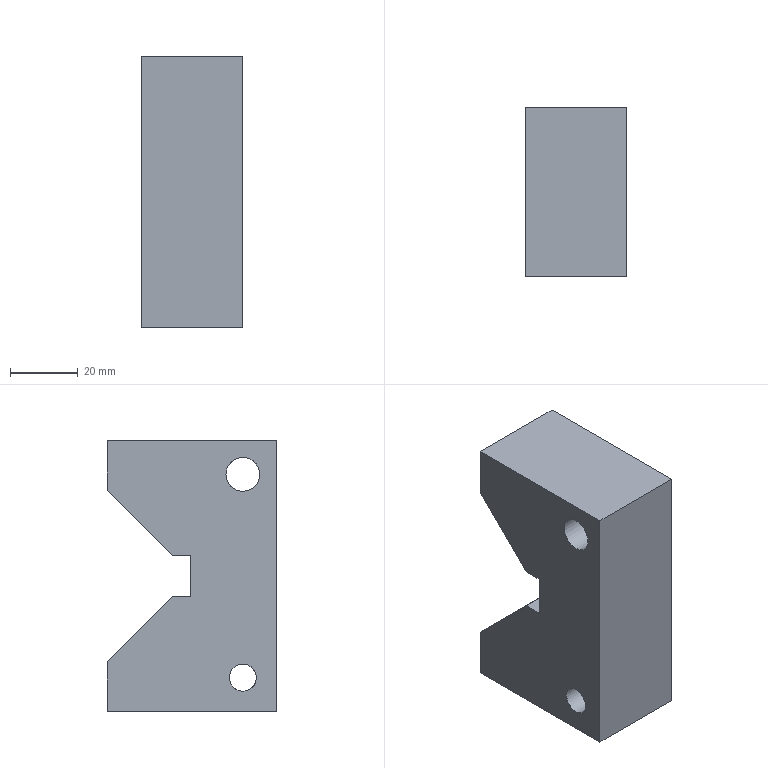Component | NX | FIXED_V_BLOCK | 1 solid | 16 faces | volume 95646 mm3 | plane 13 | cylinder 3 | commonest cylinder face diameters 10 x1 13 x1 8 x1